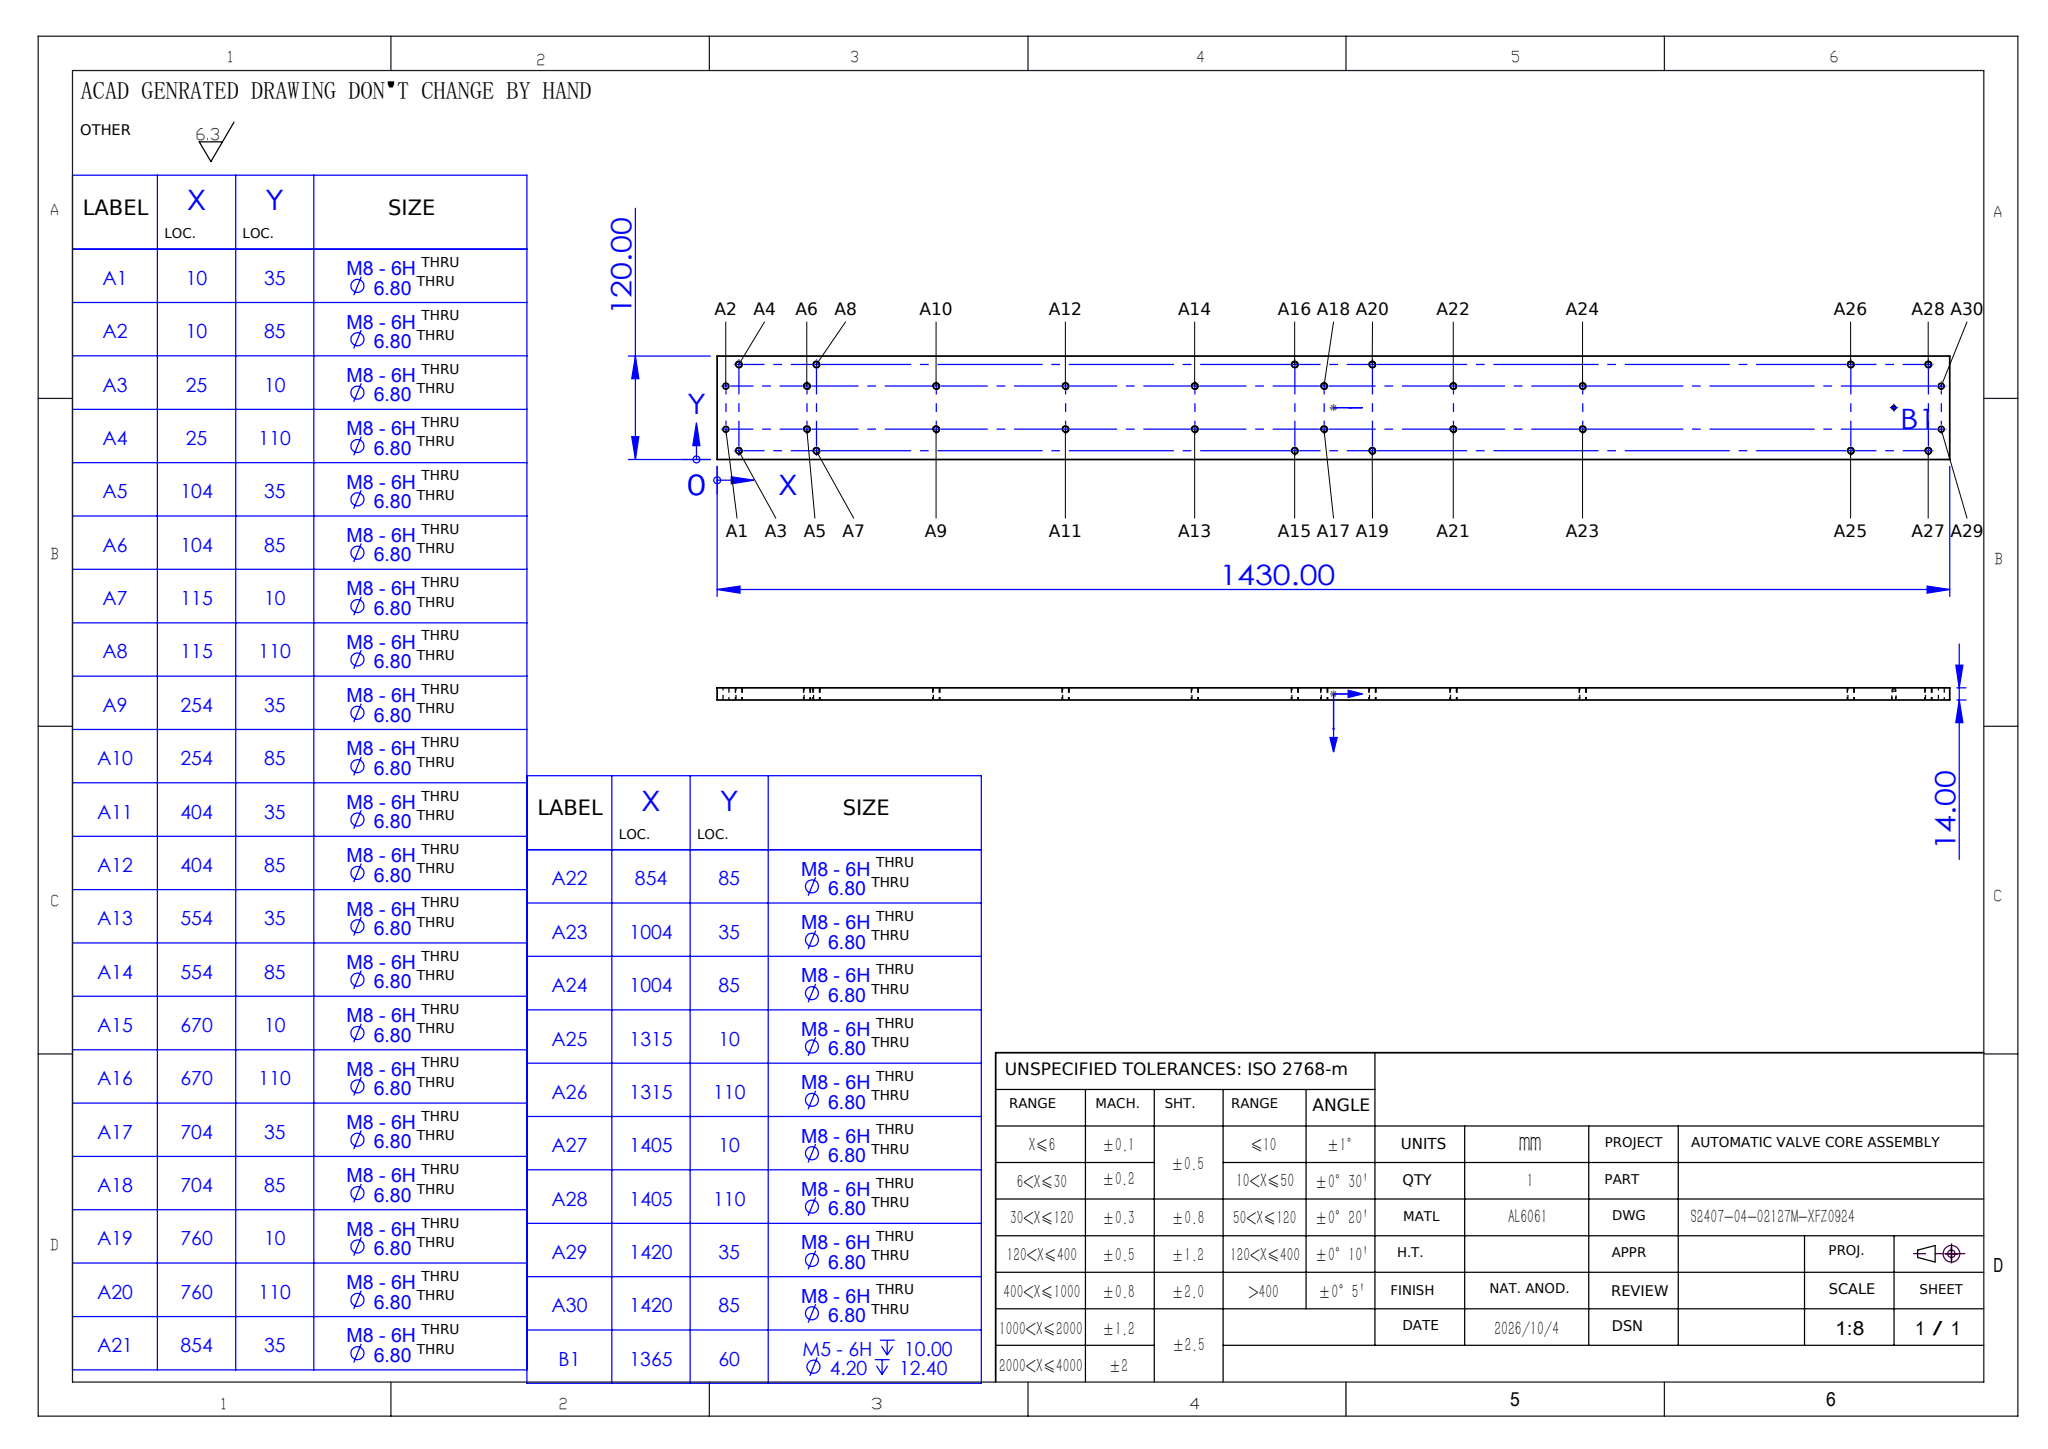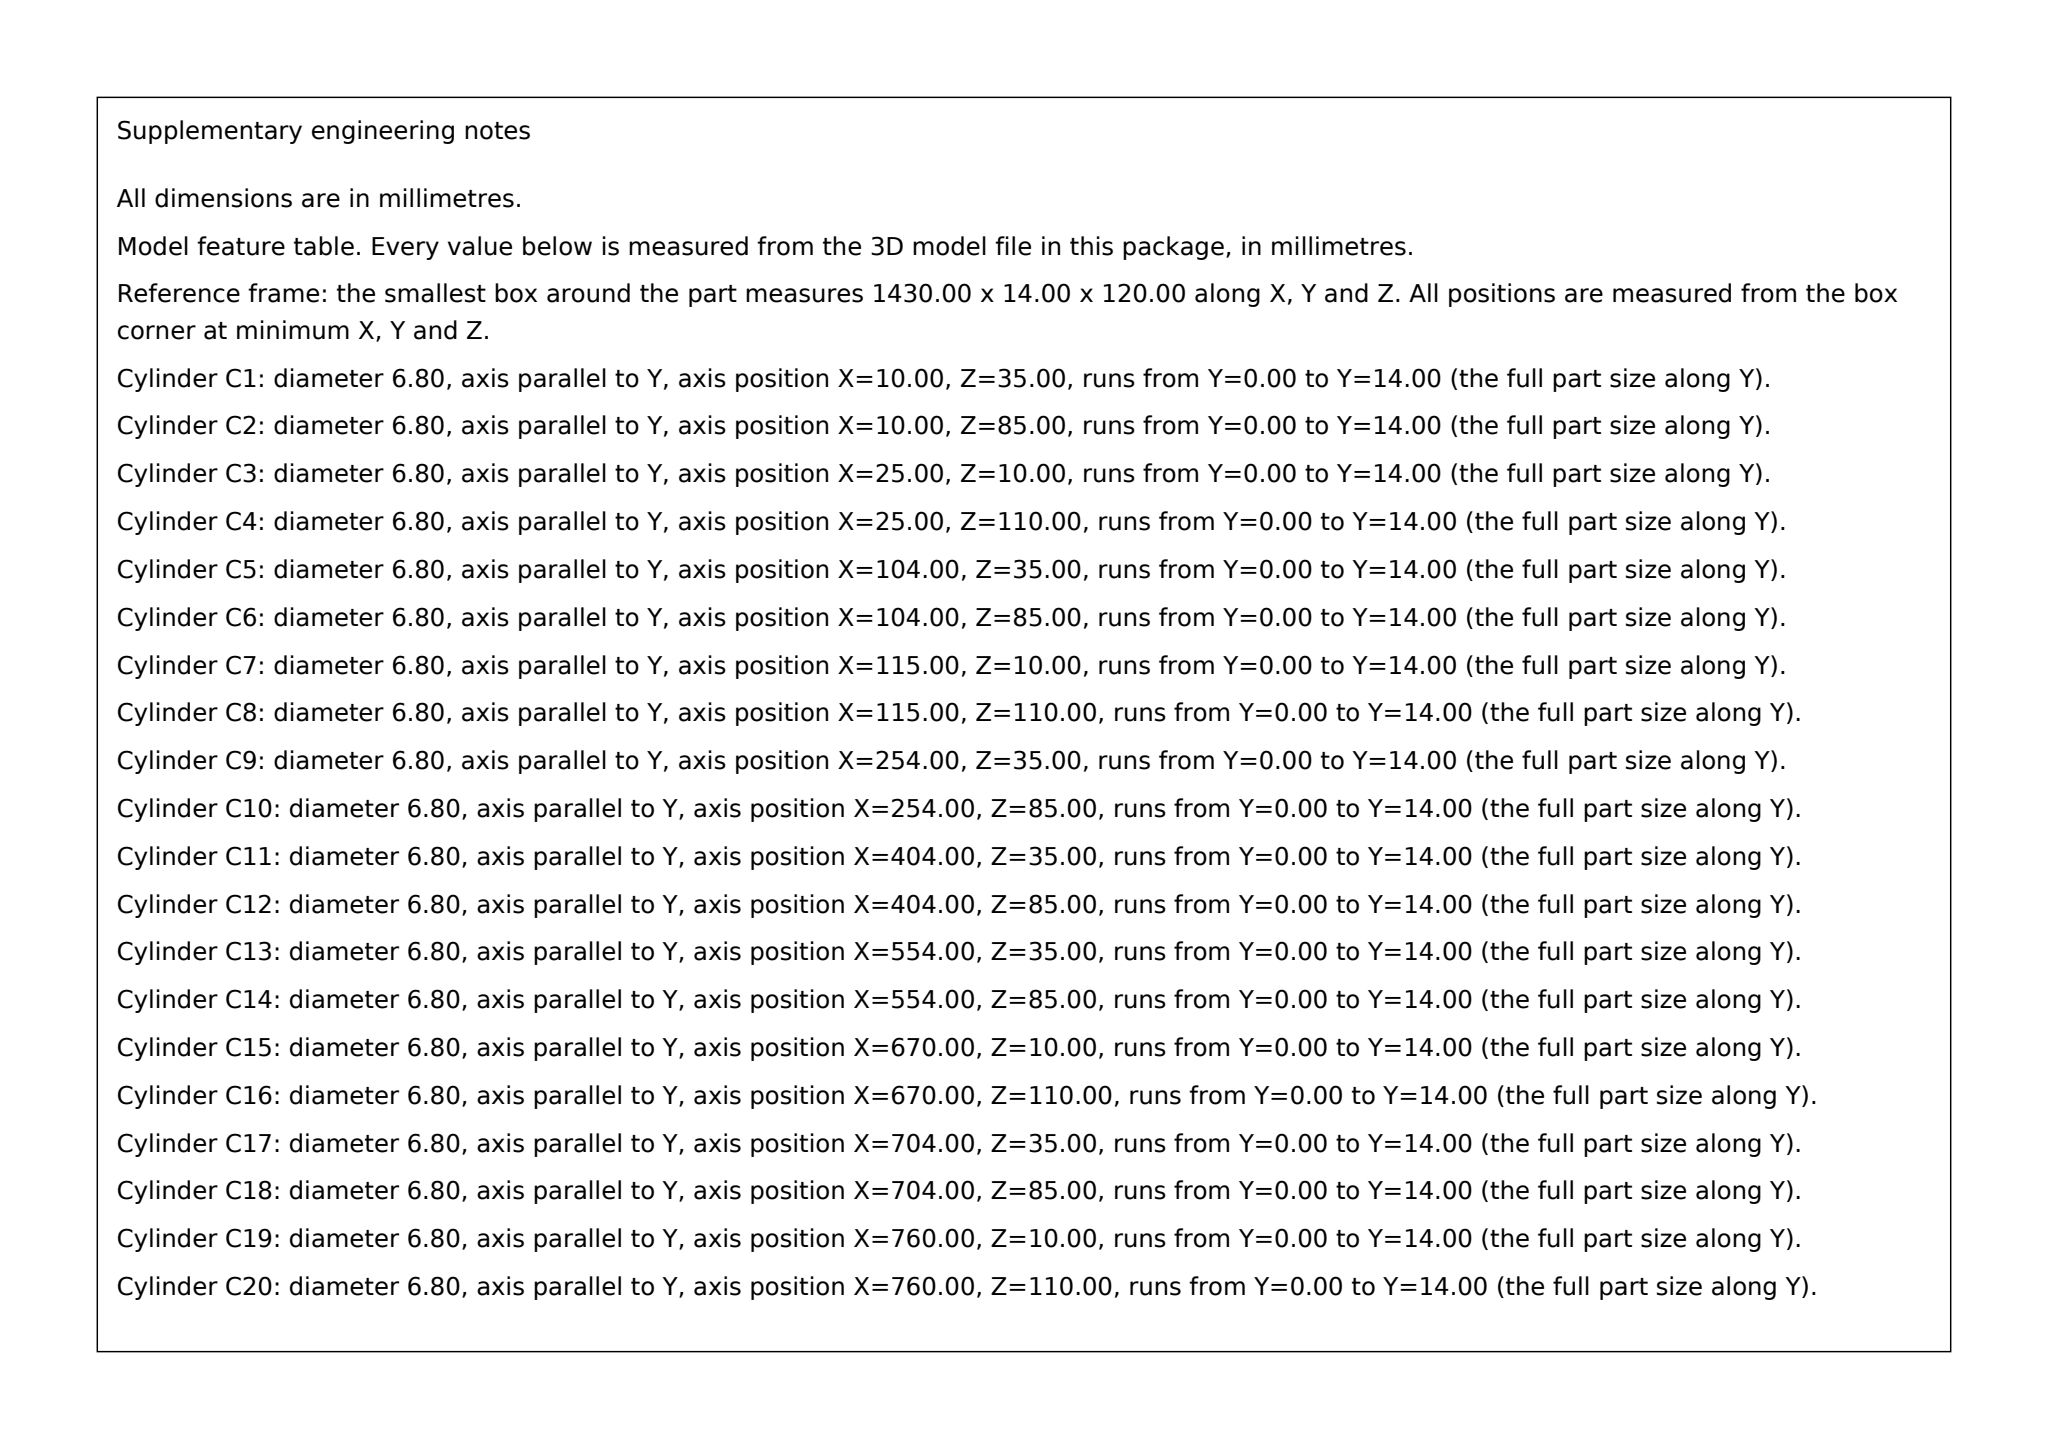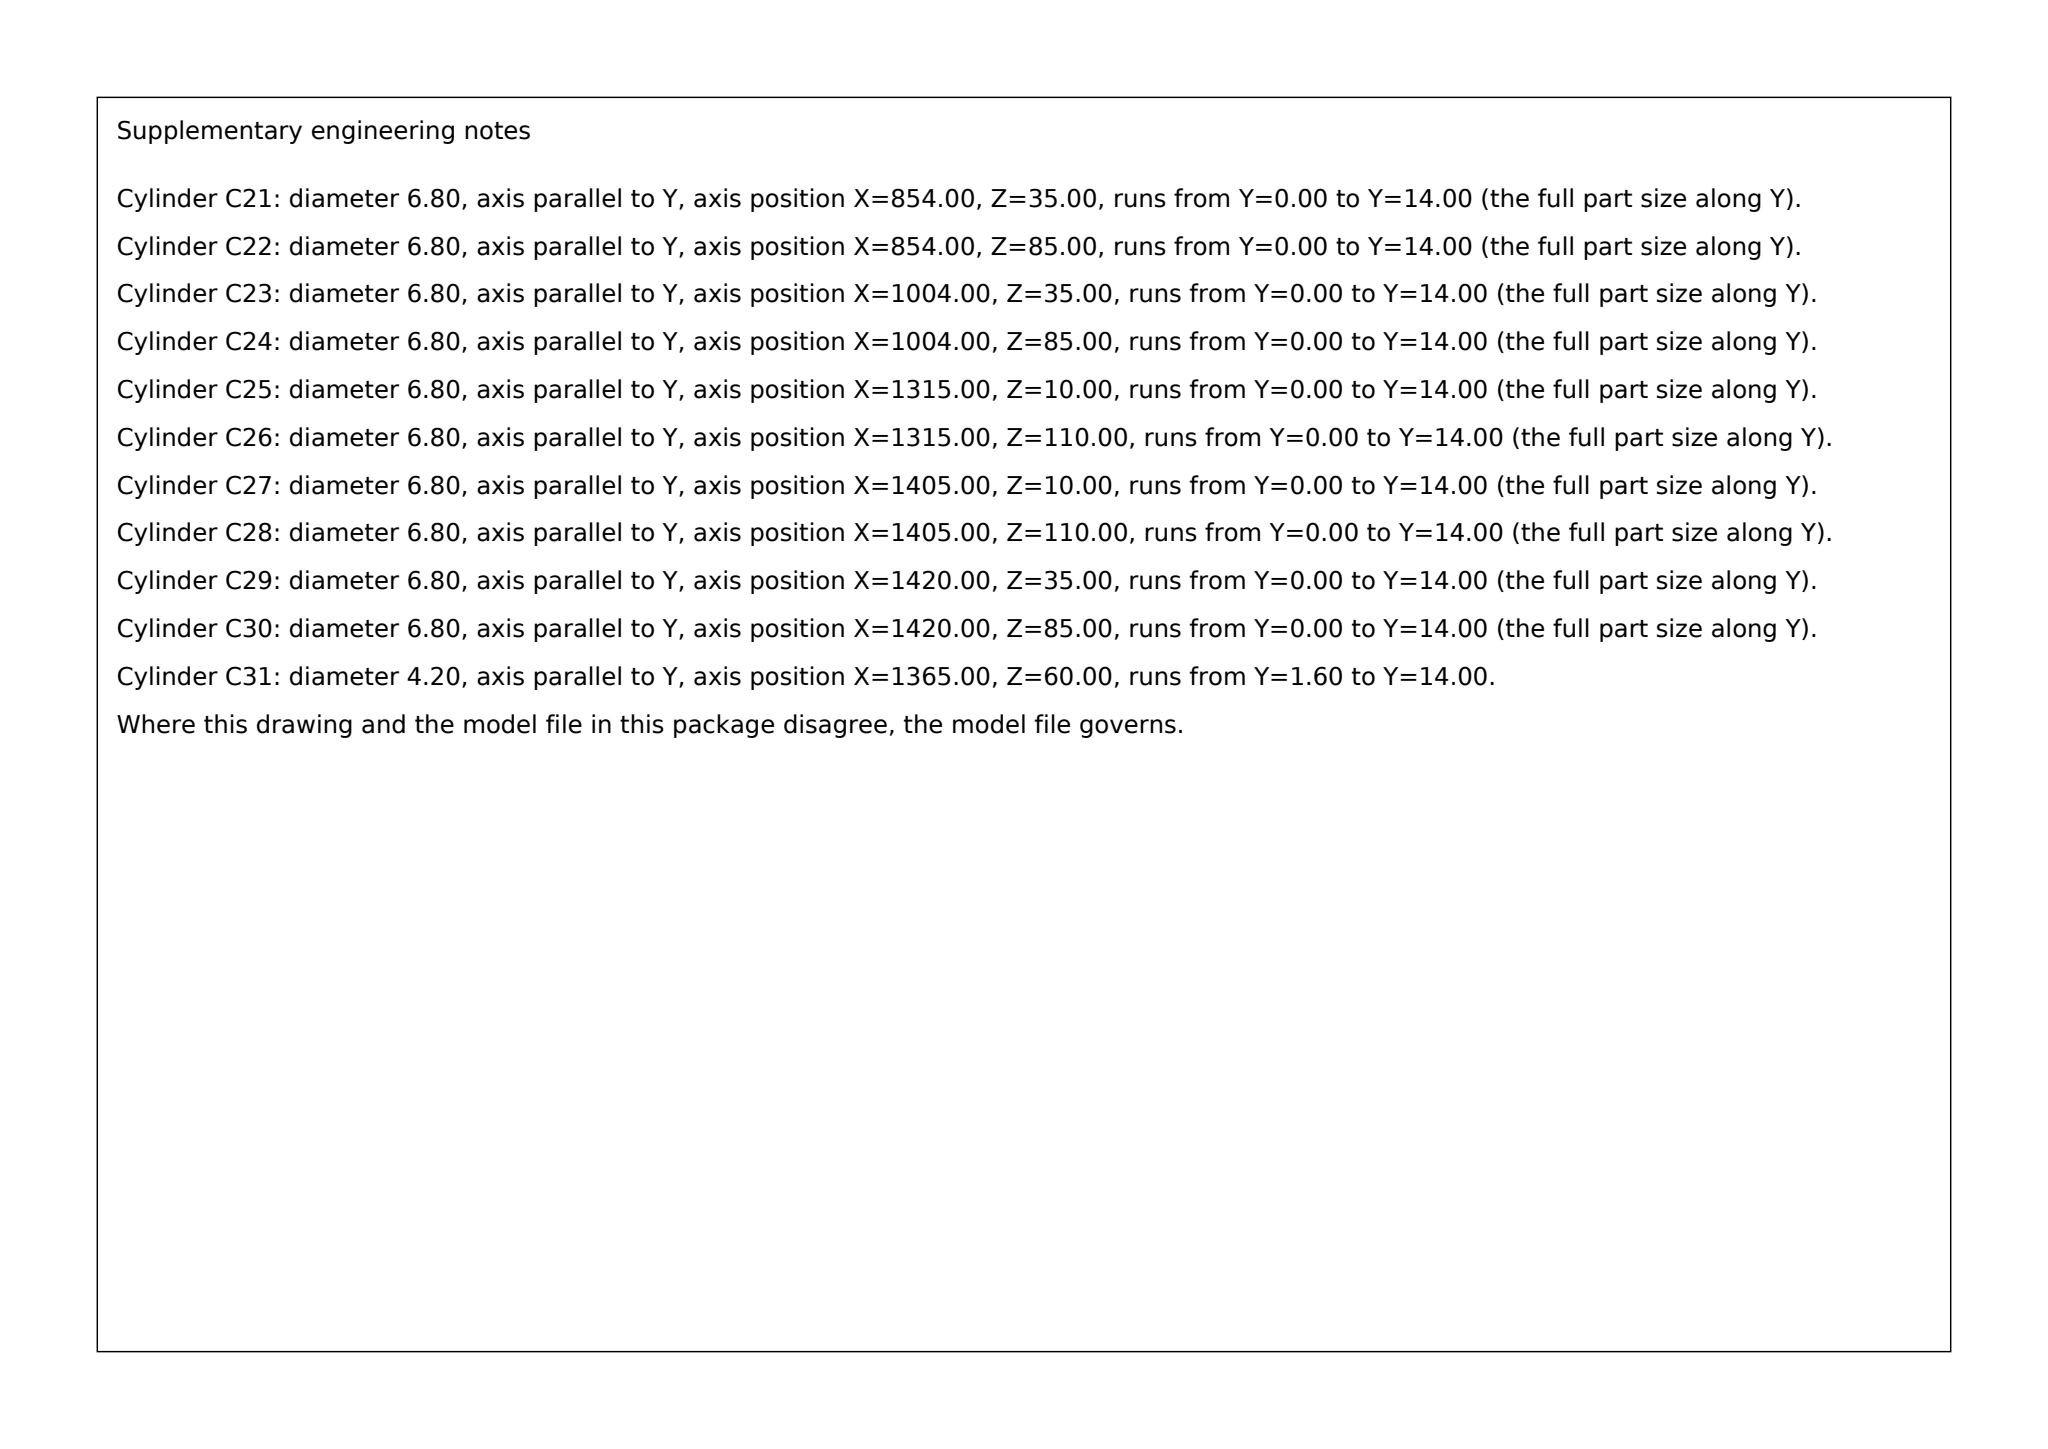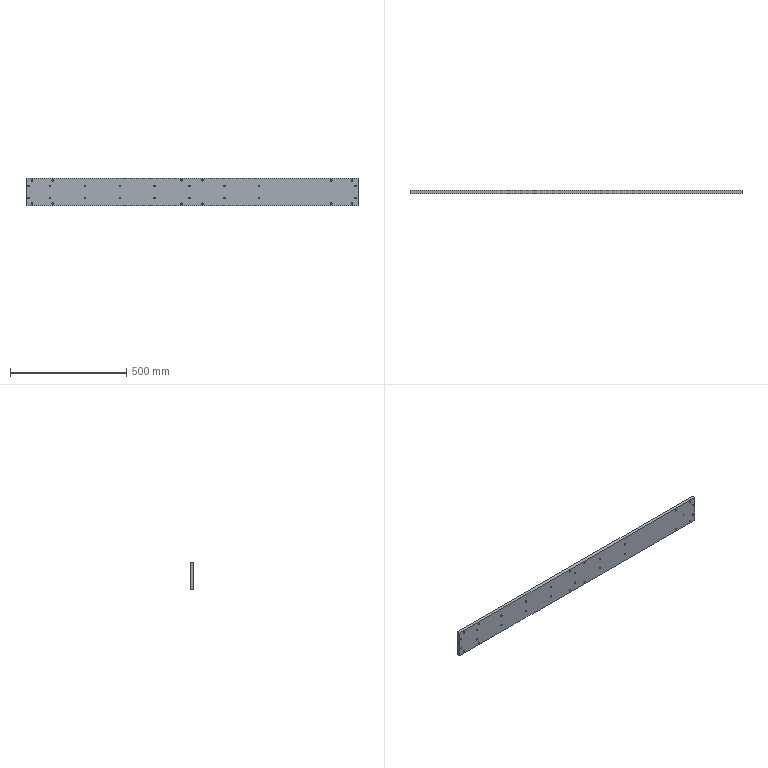Part | SolidWorks | mm | 1 solid | 70 faces | box 1430 x 14 x 120 mm | volume 2386969 mm3 | cylinder 62 | plane 6 | cone 2 | commonest cylinder face diameters 6.8 x60 4.2 x2
build123d program:
from build123d import *

# Parameters (mm, degrees)
SKETCH1_W             = 1430
SKETCH1_H             = 120
BOSS_EXTRUDE1_DEPTH   = 7
M8_TAPPED_HOLE1_D     = 6.8
M8_TAPPED_HOLE2_D     = 6.8
M5_TAPPED_HOLE1_D     = 4.2
M5_TAPPED_HOLE1_DEPTH = 12.4
M5_TAPPED_HOLE1_TIP   = 1.262


with BuildPart() as part:
    # Sketch1 → Boss-Extrude1 (new, symmetric)
    with BuildSketch(Plane(origin=(0, 0, 0), x_dir=(1, 0, 0), z_dir=(0, 1, 0))):
        Rectangle(SKETCH1_W, SKETCH1_H)
    extrude(amount=BOSS_EXTRUDE1_DEPTH, both=True)

    # M8 Tapped Hole1 (through all)
    with Locations(Plane(origin=(0, 7, 0), x_dir=(1, 0, 0), z_dir=(0, 1, 0))):
        with Locations((-690, 50), (-600, -50), (-690, -50), (-600, 50), (-45, 50), (45, -50), (-45, -50), (45, 50), (600, 50), (690, -50), (600, -50), (690, 50)):
            Hole(M8_TAPPED_HOLE1_D / 2)

    # M8 Tapped Hole2 (through all)
    with Locations(Plane(origin=(0, 7, 0), x_dir=(1, 0, 0), z_dir=(0, 1, 0))):
        with Locations((705, 25), (-611, 25), (-611, -25), (-461, 25), (-461, -25), (-311, 25), (-311, -25), (-161, 25), (-161, -25), (-11, 25), (-11, -25), (139, 25), (139, -25), (289, 25), (289, -25), (-705, -25), (-705, 25), (705, -25)):
            Hole(M8_TAPPED_HOLE2_D / 2)

    # M5 Tapped Hole1
    with Locations(Plane(origin=(0, 7, 0), x_dir=(1, 0, 0), z_dir=(0, 1, 0))):
        with Locations((650, 0)):
            Hole(M5_TAPPED_HOLE1_D / 2, depth=M5_TAPPED_HOLE1_DEPTH)
            with Locations((0, 0, -(M5_TAPPED_HOLE1_DEPTH + M5_TAPPED_HOLE1_TIP / 2))):  # 118° drill point
                Cone(0, M5_TAPPED_HOLE1_D / 2, M5_TAPPED_HOLE1_TIP, mode=Mode.SUBTRACT)


solid = part.part